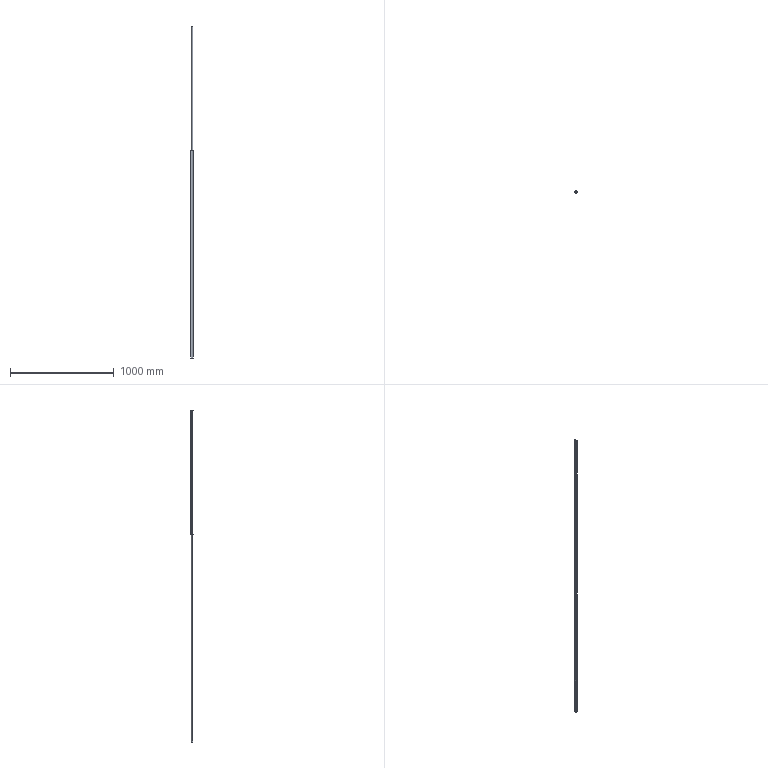Component | SolidWorks | 12ATransverseStraighteningPlatePart-2_12A10_Steel_Rib-1 | 4 solids | 16 faces | box 24 x 27 x 3200 mm | volume 723823 mm3 | cylinder 8 | plane 8 | commonest cylinder face diameters 12 x8
build123d program:
from build123d import *

# Parameters (mm, degrees)
SKETCH1_R             = 6
BOSS_EXTRUDE1_DEPTH   = 1200
BOSS_EXTRUDE1_2_DEPTH = 1200
SKETCH3_R             = 6
BOSS_EXTRUDE2_DEPTH   = 2000
SKETCH4_R             = 6
BOSS_EXTRUDE4_DEPTH   = 2000


with BuildPart() as part:
    # Sketch1 → Boss-Extrude1 (new body)
    with BuildSketch(Plane(origin=(0, 0, 0), x_dir=(1, 0, 0), z_dir=(0, 1, 0))):
        with Locations(Location((0, 0, 0), (0, 0, 270))):
            Circle(SKETCH1_R)
    extrude(amount=BOSS_EXTRUDE1_DEPTH)


with BuildPart() as body_2:
    # Sketch1 → Boss-Extrude1 2 (new body)
    with BuildSketch(Plane(origin=(0, 0, 0), x_dir=(1, 0, 0), z_dir=(0, 1, 0))):
        with Locations(Location((15, 0, 0), (0, 0, 270))):
            Circle(SKETCH1_R)
    extrude(amount=BOSS_EXTRUDE1_2_DEPTH)


with BuildPart() as body_3:
    # Sketch3 → Boss-Extrude2 (new body)
    with BuildSketch(Plane.XZ.offset(-1200)):
        with Locations(Location((7.5, -6, 0), (0, 0, 270))):
            Circle(SKETCH3_R)
    extrude(amount=-BOSS_EXTRUDE2_DEPTH)


with BuildPart() as body_4:
    # Sketch4 → Boss-Extrude4 (new body)
    with BuildSketch(Plane.XZ.offset(-1200)):
        with Locations(Location((7.5, 6, 0), (0, 0, 270))):
            Circle(SKETCH4_R)
    extrude(amount=-BOSS_EXTRUDE4_DEPTH)


solid = Compound([part.part, body_2.part, body_3.part, body_4.part])

# Placed as in the assembly
solid = solid.moved(Location((159.367, 112.46, 566), (-90, 90, 0)))
STEP:
#1=COLOUR_RGB('',0.7922,0.8196,0.9333);
#2=FILL_AREA_STYLE_COLOUR('',#1);
#3=FILL_AREA_STYLE('',(#2));
#4=SURFACE_STYLE_FILL_AREA(#3);
#5=SURFACE_SIDE_STYLE('',(#4));
#6=SURFACE_STYLE_USAGE(.BOTH.,#5);
#7=PRESENTATION_STYLE_ASSIGNMENT((#6));
#8=CARTESIAN_POINT('',(6.274,4.132,-103.701));
#9=VERTEX_POINT('',#8);
#10=CARTESIAN_POINT('',(6.747,4.132,-103.701));
#11=VERTEX_POINT('',#10);
#12=CARTESIAN_POINT('',(6.511,4.132,-103.701));
#13=DIRECTION('',(0.,0.,1.));
#14=DIRECTION('',(-1.,-0.,0.));
#15=AXIS2_PLACEMENT_3D('',#12,#13,#14);
#16=CIRCLE('',#15,0.2362);
#17=EDGE_CURVE('',#9,#11,#16,.T.);
#18=ORIENTED_EDGE('',*,*,#17,.T.);
#19=CARTESIAN_POINT('',(6.747,4.132,-24.961));
#20=VERTEX_POINT('',#19);
#21=CARTESIAN_POINT('',(6.747,4.132,-103.701));
#22=DIRECTION('',(0.,0.,1.));
#23=VECTOR('',#22,39.37);
#24=LINE('',#21,#23);
#25=EDGE_CURVE('',#11,#20,#24,.T.);
#26=ORIENTED_EDGE('',*,*,#25,.T.);
#27=CARTESIAN_POINT('',(6.274,4.132,-24.961));
#28=VERTEX_POINT('',#27);
#29=CARTESIAN_POINT('',(6.511,4.132,-24.961));
#30=DIRECTION('',(0.,0.,1.));
#31=DIRECTION('',(-1.,-0.,0.));
#32=AXIS2_PLACEMENT_3D('',#29,#30,#31);
#33=CIRCLE('',#32,0.2362);
#34=EDGE_CURVE('',#28,#20,#33,.T.);
#35=ORIENTED_EDGE('',*,*,#34,.F.);
#36=CARTESIAN_POINT('',(6.274,4.132,-103.701));
#37=DIRECTION('',(0.,0.,1.));
#38=VECTOR('',#37,39.37);
#39=LINE('',#36,#38);
#40=EDGE_CURVE('',#9,#28,#39,.T.);
#41=ORIENTED_EDGE('',*,*,#40,.F.);
#42=EDGE_LOOP('',(#18,#26,#35,#41));
#43=FACE_OUTER_BOUND('',#42,.T.);
#44=CARTESIAN_POINT('',(6.511,4.132,-103.701));
#45=DIRECTION('',(0.,0.,1.));
#46=DIRECTION('',(-1.,-0.,0.));
#47=AXIS2_PLACEMENT_3D('',#44,#45,#46);
#48=CYLINDRICAL_SURFACE('',#47,0.2362);
#49=ADVANCED_FACE('',(#43),#48,.T.);
#50=ORIENTED_EDGE('',*,*,#25,.F.);
#51=CARTESIAN_POINT('',(6.511,4.132,-103.701));
#52=DIRECTION('',(0.,0.,1.));
#53=DIRECTION('',(-1.,-0.,0.));
#54=AXIS2_PLACEMENT_3D('',#51,#52,#53);
#55=CIRCLE('',#54,0.2362);
#56=EDGE_CURVE('',#11,#9,#55,.T.);
#57=ORIENTED_EDGE('',*,*,#56,.T.);
#58=ORIENTED_EDGE('',*,*,#40,.T.);
#59=CARTESIAN_POINT('',(6.511,4.132,-24.961));
#60=DIRECTION('',(0.,0.,1.));
#61=DIRECTION('',(-1.,-0.,0.));
#62=AXIS2_PLACEMENT_3D('',#59,#60,#61);
#63=CIRCLE('',#62,0.2362);
#64=EDGE_CURVE('',#20,#28,#63,.T.);
#65=ORIENTED_EDGE('',*,*,#64,.F.);
#66=EDGE_LOOP('',(#50,#57,#58,#65));
#67=FACE_OUTER_BOUND('',#66,.T.);
#68=CARTESIAN_POINT('',(6.511,4.132,-103.701));
#69=DIRECTION('',(0.,0.,1.));
#70=DIRECTION('',(-1.,-0.,0.));
#71=AXIS2_PLACEMENT_3D('',#68,#69,#70);
#72=CYLINDRICAL_SURFACE('',#71,0.2362);
#73=ADVANCED_FACE('',(#67),#72,.T.);
#74=ORIENTED_EDGE('',*,*,#17,.F.);
#75=ORIENTED_EDGE('',*,*,#56,.F.);
#76=EDGE_LOOP('',(#74,#75));
#77=FACE_OUTER_BOUND('',#76,.T.);
#78=CARTESIAN_POINT('',(6.511,4.132,-103.701));
#79=DIRECTION('',(0.,0.,1.));
#80=DIRECTION('',(-1.,-0.,0.));
#81=AXIS2_PLACEMENT_3D('',#78,#79,#80);
#82=PLANE('',#81);
#83=ADVANCED_FACE('',(#77),#82,.F.);
#84=ORIENTED_EDGE('',*,*,#34,.T.);
#85=ORIENTED_EDGE('',*,*,#64,.T.);
#86=EDGE_LOOP('',(#84,#85));
#87=FACE_OUTER_BOUND('',#86,.T.);
#88=CARTESIAN_POINT('',(6.511,4.132,-24.961));
#89=DIRECTION('',(0.,0.,1.));
#90=DIRECTION('',(-1.,-0.,0.));
#91=AXIS2_PLACEMENT_3D('',#88,#89,#90);
#92=PLANE('',#91);
#93=ADVANCED_FACE('',(#87),#92,.T.);
#94=CLOSED_SHELL('',(#49,#73,#83,#93));
#95=MANIFOLD_SOLID_BREP('',#94);
#96=STYLED_ITEM('',(#7),#95);
#97=(LENGTH_UNIT()NAMED_UNIT(*)SI_UNIT($,.METRE.));
#98=LENGTH_MEASURE_WITH_UNIT(LENGTH_MEASURE(0.0254),#97);
#99=DIMENSIONAL_EXPONENTS(1.,0.,0.,0.,0.,0.,0.);
#100=(CONVERSION_BASED_UNIT('',#98)LENGTH_UNIT()NAMED_UNIT(#99));
#101=UNCERTAINTY_MEASURE_WITH_UNIT(LENGTH_MEASURE(0.00001),#100,'','');
#102=(NAMED_UNIT(*)PLANE_ANGLE_UNIT()SI_UNIT($,.RADIAN.));
#103=(NAMED_UNIT(*)SI_UNIT($,.STERADIAN.)SOLID_ANGLE_UNIT());
#104=(GEOMETRIC_REPRESENTATION_CONTEXT(3)GLOBAL_UNCERTAINTY_ASSIGNED_CONTEXT((#101))GLOBAL_UNIT_ASSIGNED_CONTEXT((#100,#102,#103))REPRESENTATION_CONTEXT('',''));
#105=MECHANICAL_DESIGN_GEOMETRIC_PRESENTATION_REPRESENTATION('',(#96),#104);
#106=COLOUR_RGB('',0.7922,0.8196,0.9333);
#107=FILL_AREA_STYLE_COLOUR('',#106);
#108=FILL_AREA_STYLE('',(#107));
#109=SURFACE_STYLE_FILL_AREA(#108);
#110=SURFACE_SIDE_STYLE('',(#109));
#111=SURFACE_STYLE_USAGE(.BOTH.,#110);
#112=PRESENTATION_STYLE_ASSIGNMENT((#111));
#113=CARTESIAN_POINT('',(5.802,4.132,-103.701));
#114=VERTEX_POINT('',#113);
#115=CARTESIAN_POINT('',(6.274,4.132,-103.701));
#116=VERTEX_POINT('',#115);
#117=CARTESIAN_POINT('',(6.038,4.132,-103.701));
#118=DIRECTION('',(0.,0.,1.));
#119=DIRECTION('',(-1.,-0.,0.));
#120=AXIS2_PLACEMENT_3D('',#117,#118,#119);
#121=CIRCLE('',#120,0.2362);
#122=EDGE_CURVE('',#114,#116,#121,.T.);
#123=ORIENTED_EDGE('',*,*,#122,.T.);
#124=CARTESIAN_POINT('',(6.274,4.132,-24.961));
#125=VERTEX_POINT('',#124);
#126=CARTESIAN_POINT('',(6.274,4.132,-103.701));
#127=DIRECTION('',(0.,0.,1.));
#128=VECTOR('',#127,39.37);
#129=LINE('',#126,#128);
#130=EDGE_CURVE('',#116,#125,#129,.T.);
#131=ORIENTED_EDGE('',*,*,#130,.T.);
#132=CARTESIAN_POINT('',(5.802,4.132,-24.961));
#133=VERTEX_POINT('',#132);
#134=CARTESIAN_POINT('',(6.038,4.132,-24.961));
#135=DIRECTION('',(0.,0.,1.));
#136=DIRECTION('',(-1.,-0.,0.));
#137=AXIS2_PLACEMENT_3D('',#134,#135,#136);
#138=CIRCLE('',#137,0.2362);
#139=EDGE_CURVE('',#133,#125,#138,.T.);
#140=ORIENTED_EDGE('',*,*,#139,.F.);
#141=CARTESIAN_POINT('',(5.802,4.132,-103.701));
#142=DIRECTION('',(0.,0.,1.));
#143=VECTOR('',#142,39.37);
#144=LINE('',#141,#143);
#145=EDGE_CURVE('',#114,#133,#144,.T.);
#146=ORIENTED_EDGE('',*,*,#145,.F.);
#147=EDGE_LOOP('',(#123,#131,#140,#146));
#148=FACE_OUTER_BOUND('',#147,.T.);
#149=CARTESIAN_POINT('',(6.038,4.132,-103.701));
#150=DIRECTION('',(0.,0.,1.));
#151=DIRECTION('',(-1.,-0.,0.));
#152=AXIS2_PLACEMENT_3D('',#149,#150,#151);
#153=CYLINDRICAL_SURFACE('',#152,0.2362);
#154=ADVANCED_FACE('',(#148),#153,.T.);
#155=ORIENTED_EDGE('',*,*,#130,.F.);
#156=CARTESIAN_POINT('',(6.038,4.132,-103.701));
#157=DIRECTION('',(0.,0.,1.));
#158=DIRECTION('',(-1.,-0.,0.));
#159=AXIS2_PLACEMENT_3D('',#156,#157,#158);
#160=CIRCLE('',#159,0.2362);
#161=EDGE_CURVE('',#116,#114,#160,.T.);
#162=ORIENTED_EDGE('',*,*,#161,.T.);
#163=ORIENTED_EDGE('',*,*,#145,.T.);
#164=CARTESIAN_POINT('',(6.038,4.132,-24.961));
#165=DIRECTION('',(0.,0.,1.));
#166=DIRECTION('',(-1.,-0.,0.));
#167=AXIS2_PLACEMENT_3D('',#164,#165,#166);
#168=CIRCLE('',#167,0.2362);
#169=EDGE_CURVE('',#125,#133,#168,.T.);
#170=ORIENTED_EDGE('',*,*,#169,.F.);
#171=EDGE_LOOP('',(#155,#162,#163,#170));
#172=FACE_OUTER_BOUND('',#171,.T.);
#173=CARTESIAN_POINT('',(6.038,4.132,-103.701));
#174=DIRECTION('',(0.,0.,1.));
#175=DIRECTION('',(-1.,-0.,0.));
#176=AXIS2_PLACEMENT_3D('',#173,#174,#175);
#177=CYLINDRICAL_SURFACE('',#176,0.2362);
#178=ADVANCED_FACE('',(#172),#177,.T.);
#179=ORIENTED_EDGE('',*,*,#122,.F.);
#180=ORIENTED_EDGE('',*,*,#161,.F.);
#181=EDGE_LOOP('',(#179,#180));
#182=FACE_OUTER_BOUND('',#181,.T.);
#183=CARTESIAN_POINT('',(6.038,4.132,-103.701));
#184=DIRECTION('',(0.,0.,1.));
#185=DIRECTION('',(-1.,-0.,0.));
#186=AXIS2_PLACEMENT_3D('',#183,#184,#185);
#187=PLANE('',#186);
#188=ADVANCED_FACE('',(#182),#187,.F.);
#189=ORIENTED_EDGE('',*,*,#139,.T.);
#190=ORIENTED_EDGE('',*,*,#169,.T.);
#191=EDGE_LOOP('',(#189,#190));
#192=FACE_OUTER_BOUND('',#191,.T.);
#193=CARTESIAN_POINT('',(6.038,4.132,-24.961));
#194=DIRECTION('',(0.,0.,1.));
#195=DIRECTION('',(-1.,-0.,0.));
#196=AXIS2_PLACEMENT_3D('',#193,#194,#195);
#197=PLANE('',#196);
#198=ADVANCED_FACE('',(#192),#197,.T.);
#199=CLOSED_SHELL('',(#154,#178,#188,#198));
#200=MANIFOLD_SOLID_BREP('',#199);
#201=STYLED_ITEM('',(#112),#200);
#202=PRESENTATION_LAYER_ASSIGNMENT('','',(#201));
#203=(LENGTH_UNIT()NAMED_UNIT(*)SI_UNIT($,.METRE.));
#204=LENGTH_MEASURE_WITH_UNIT(LENGTH_MEASURE(0.0254),#203);
#205=DIMENSIONAL_EXPONENTS(1.,0.,0.,0.,0.,0.,0.);
#206=(CONVERSION_BASED_UNIT('',#204)LENGTH_UNIT()NAMED_UNIT(#205));
#207=UNCERTAINTY_MEASURE_WITH_UNIT(LENGTH_MEASURE(0.00001),#206,'','');
#208=(NAMED_UNIT(*)PLANE_ANGLE_UNIT()SI_UNIT($,.RADIAN.));
#209=(NAMED_UNIT(*)SI_UNIT($,.STERADIAN.)SOLID_ANGLE_UNIT());
#210=(GEOMETRIC_REPRESENTATION_CONTEXT(3)GLOBAL_UNCERTAINTY_ASSIGNED_CONTEXT((#207))GLOBAL_UNIT_ASSIGNED_CONTEXT((#206,#208,#209))REPRESENTATION_CONTEXT('',''));
#211=MECHANICAL_DESIGN_GEOMETRIC_PRESENTATION_REPRESENTATION('',(#201),#210);
#212=COLOUR_RGB('',0.7922,0.8196,0.9333);
#213=FILL_AREA_STYLE_COLOUR('',#212);
#214=FILL_AREA_STYLE('',(#213));
#215=SURFACE_STYLE_FILL_AREA(#214);
#216=SURFACE_SIDE_STYLE('',(#215));
#217=SURFACE_STYLE_USAGE(.BOTH.,#216);
#218=PRESENTATION_STYLE_ASSIGNMENT((#217));
#219=CARTESIAN_POINT('',(6.511,4.428,-24.961));
#220=VERTEX_POINT('',#219);
#221=CARTESIAN_POINT('',(6.038,4.428,-24.961));
#222=VERTEX_POINT('',#221);
#223=CARTESIAN_POINT('',(6.274,4.428,-24.961));
#224=DIRECTION('',(-0.,-0.,-1.));
#225=DIRECTION('',(1.,0.,0.));
#226=AXIS2_PLACEMENT_3D('',#223,#224,#225);
#227=CIRCLE('',#226,0.2362);
#228=EDGE_CURVE('',#220,#222,#227,.T.);
#229=ORIENTED_EDGE('',*,*,#228,.F.);
#230=CARTESIAN_POINT('',(6.511,4.428,22.283));
#231=VERTEX_POINT('',#230);
#232=CARTESIAN_POINT('',(6.511,4.428,-24.961));
#233=DIRECTION('',(0.,0.,1.));
#234=VECTOR('',#233,39.37);
#235=LINE('',#232,#234);
#236=EDGE_CURVE('',#220,#231,#235,.T.);
#237=ORIENTED_EDGE('',*,*,#236,.T.);
#238=CARTESIAN_POINT('',(6.038,4.428,22.283));
#239=VERTEX_POINT('',#238);
#240=CARTESIAN_POINT('',(6.274,4.428,22.283));
#241=DIRECTION('',(-0.,-0.,-1.));
#242=DIRECTION('',(1.,0.,0.));
#243=AXIS2_PLACEMENT_3D('',#240,#241,#242);
#244=CIRCLE('',#243,0.2362);
#245=EDGE_CURVE('',#231,#239,#244,.T.);
#246=ORIENTED_EDGE('',*,*,#245,.T.);
#247=CARTESIAN_POINT('',(6.038,4.428,-24.961));
#248=DIRECTION('',(0.,0.,1.));
#249=VECTOR('',#248,39.37);
#250=LINE('',#247,#249);
#251=EDGE_CURVE('',#222,#239,#250,.T.);
#252=ORIENTED_EDGE('',*,*,#251,.F.);
#253=EDGE_LOOP('',(#229,#237,#246,#252));
#254=FACE_OUTER_BOUND('',#253,.T.);
#255=CARTESIAN_POINT('',(6.274,4.428,-24.961));
#256=DIRECTION('',(0.,0.,1.));
#257=DIRECTION('',(-1.,-0.,0.));
#258=AXIS2_PLACEMENT_3D('',#255,#256,#257);
#259=CYLINDRICAL_SURFACE('',#258,0.2362);
#260=ADVANCED_FACE('',(#254),#259,.T.);
#261=ORIENTED_EDGE('',*,*,#236,.F.);
#262=CARTESIAN_POINT('',(6.274,4.428,-24.961));
#263=DIRECTION('',(-0.,-0.,-1.));
#264=DIRECTION('',(1.,0.,0.));
#265=AXIS2_PLACEMENT_3D('',#262,#263,#264);
#266=CIRCLE('',#265,0.2362);
#267=EDGE_CURVE('',#222,#220,#266,.T.);
#268=ORIENTED_EDGE('',*,*,#267,.F.);
#269=ORIENTED_EDGE('',*,*,#251,.T.);
#270=CARTESIAN_POINT('',(6.274,4.428,22.283));
#271=DIRECTION('',(-0.,-0.,-1.));
#272=DIRECTION('',(1.,0.,0.));
#273=AXIS2_PLACEMENT_3D('',#270,#271,#272);
#274=CIRCLE('',#273,0.2362);
#275=EDGE_CURVE('',#239,#231,#274,.T.);
#276=ORIENTED_EDGE('',*,*,#275,.T.);
#277=EDGE_LOOP('',(#261,#268,#269,#276));
#278=FACE_OUTER_BOUND('',#277,.T.);
#279=CARTESIAN_POINT('',(6.274,4.428,-24.961));
#280=DIRECTION('',(0.,0.,1.));
#281=DIRECTION('',(-1.,-0.,0.));
#282=AXIS2_PLACEMENT_3D('',#279,#280,#281);
#283=CYLINDRICAL_SURFACE('',#282,0.2362);
#284=ADVANCED_FACE('',(#278),#283,.T.);
#285=ORIENTED_EDGE('',*,*,#267,.T.);
#286=ORIENTED_EDGE('',*,*,#228,.T.);
#287=EDGE_LOOP('',(#285,#286));
#288=FACE_OUTER_BOUND('',#287,.T.);
#289=CARTESIAN_POINT('',(6.274,4.428,-24.961));
#290=DIRECTION('',(-0.,-0.,-1.));
#291=DIRECTION('',(1.,0.,-0.));
#292=AXIS2_PLACEMENT_3D('',#289,#290,#291);
#293=PLANE('',#292);
#294=ADVANCED_FACE('',(#288),#293,.T.);
#295=ORIENTED_EDGE('',*,*,#275,.F.);
#296=ORIENTED_EDGE('',*,*,#245,.F.);
#297=EDGE_LOOP('',(#295,#296));
#298=FACE_OUTER_BOUND('',#297,.T.);
#299=CARTESIAN_POINT('',(6.274,4.428,22.283));
#300=DIRECTION('',(-0.,-0.,-1.));
#301=DIRECTION('',(1.,0.,-0.));
#302=AXIS2_PLACEMENT_3D('',#299,#300,#301);
#303=PLANE('',#302);
#304=ADVANCED_FACE('',(#298),#303,.F.);
#305=CLOSED_SHELL('',(#260,#284,#294,#304));
#306=MANIFOLD_SOLID_BREP('',#305);
#307=STYLED_ITEM('',(#218),#306);
#308=(LENGTH_UNIT()NAMED_UNIT(*)SI_UNIT($,.METRE.));
#309=LENGTH_MEASURE_WITH_UNIT(LENGTH_MEASURE(0.0254),#308);
#310=DIMENSIONAL_EXPONENTS(1.,0.,0.,0.,0.,0.,0.);
#311=(CONVERSION_BASED_UNIT('',#309)LENGTH_UNIT()NAMED_UNIT(#310));
#312=UNCERTAINTY_MEASURE_WITH_UNIT(LENGTH_MEASURE(0.00001),#311,'','');
#313=(NAMED_UNIT(*)PLANE_ANGLE_UNIT()SI_UNIT($,.RADIAN.));
#314=(NAMED_UNIT(*)SI_UNIT($,.STERADIAN.)SOLID_ANGLE_UNIT());
#315=(GEOMETRIC_REPRESENTATION_CONTEXT(3)GLOBAL_UNCERTAINTY_ASSIGNED_CONTEXT((#312))GLOBAL_UNIT_ASSIGNED_CONTEXT((#311,#313,#314))REPRESENTATION_CONTEXT('',''));
#316=MECHANICAL_DESIGN_GEOMETRIC_PRESENTATION_REPRESENTATION('',(#307),#315);
#317=PRESENTATION_LAYER_ASSIGNMENT('','',(#96));
#318=COLOUR_RGB('',0.7922,0.8196,0.9333);
#319=FILL_AREA_STYLE_COLOUR('',#318);
#320=FILL_AREA_STYLE('',(#319));
#321=SURFACE_STYLE_FILL_AREA(#320);
#322=SURFACE_SIDE_STYLE('',(#321));
#323=SURFACE_STYLE_USAGE(.BOTH.,#322);
#324=PRESENTATION_STYLE_ASSIGNMENT((#323));
#325=CARTESIAN_POINT('',(6.511,3.837,-24.961));
#326=VERTEX_POINT('',#325);
#327=CARTESIAN_POINT('',(6.038,3.837,-24.961));
#328=VERTEX_POINT('',#327);
#329=CARTESIAN_POINT('',(6.274,3.837,-24.961));
#330=DIRECTION('',(-0.,-0.,-1.));
#331=DIRECTION('',(1.,0.,0.));
#332=AXIS2_PLACEMENT_3D('',#329,#330,#331);
#333=CIRCLE('',#332,0.2362);
#334=EDGE_CURVE('',#326,#328,#333,.T.);
#335=ORIENTED_EDGE('',*,*,#334,.F.);
#336=CARTESIAN_POINT('',(6.511,3.837,22.283));
#337=VERTEX_POINT('',#336);
#338=CARTESIAN_POINT('',(6.511,3.837,-24.961));
#339=DIRECTION('',(0.,0.,1.));
#340=VECTOR('',#339,39.37);
#341=LINE('',#338,#340);
#342=EDGE_CURVE('',#326,#337,#341,.T.);
#343=ORIENTED_EDGE('',*,*,#342,.T.);
#344=CARTESIAN_POINT('',(6.038,3.837,22.283));
#345=VERTEX_POINT('',#344);
#346=CARTESIAN_POINT('',(6.274,3.837,22.283));
#347=DIRECTION('',(-0.,-0.,-1.));
#348=DIRECTION('',(1.,0.,0.));
#349=AXIS2_PLACEMENT_3D('',#346,#347,#348);
#350=CIRCLE('',#349,0.2362);
#351=EDGE_CURVE('',#337,#345,#350,.T.);
#352=ORIENTED_EDGE('',*,*,#351,.T.);
#353=CARTESIAN_POINT('',(6.038,3.837,-24.961));
#354=DIRECTION('',(0.,0.,1.));
#355=VECTOR('',#354,39.37);
#356=LINE('',#353,#355);
#357=EDGE_CURVE('',#328,#345,#356,.T.);
#358=ORIENTED_EDGE('',*,*,#357,.F.);
#359=EDGE_LOOP('',(#335,#343,#352,#358));
#360=FACE_OUTER_BOUND('',#359,.T.);
#361=CARTESIAN_POINT('',(6.274,3.837,-24.961));
#362=DIRECTION('',(0.,0.,1.));
#363=DIRECTION('',(-1.,-0.,0.));
#364=AXIS2_PLACEMENT_3D('',#361,#362,#363);
#365=CYLINDRICAL_SURFACE('',#364,0.2362);
#366=ADVANCED_FACE('',(#360),#365,.T.);
#367=ORIENTED_EDGE('',*,*,#342,.F.);
#368=CARTESIAN_POINT('',(6.274,3.837,-24.961));
#369=DIRECTION('',(-0.,-0.,-1.));
#370=DIRECTION('',(1.,0.,0.));
#371=AXIS2_PLACEMENT_3D('',#368,#369,#370);
#372=CIRCLE('',#371,0.2362);
#373=EDGE_CURVE('',#328,#326,#372,.T.);
#374=ORIENTED_EDGE('',*,*,#373,.F.);
#375=ORIENTED_EDGE('',*,*,#357,.T.);
#376=CARTESIAN_POINT('',(6.274,3.837,22.283));
#377=DIRECTION('',(-0.,-0.,-1.));
#378=DIRECTION('',(1.,0.,0.));
#379=AXIS2_PLACEMENT_3D('',#376,#377,#378);
#380=CIRCLE('',#379,0.2362);
#381=EDGE_CURVE('',#345,#337,#380,.T.);
#382=ORIENTED_EDGE('',*,*,#381,.T.);
#383=EDGE_LOOP('',(#367,#374,#375,#382));
#384=FACE_OUTER_BOUND('',#383,.T.);
#385=CARTESIAN_POINT('',(6.274,3.837,-24.961));
#386=DIRECTION('',(0.,0.,1.));
#387=DIRECTION('',(-1.,-0.,0.));
#388=AXIS2_PLACEMENT_3D('',#385,#386,#387);
#389=CYLINDRICAL_SURFACE('',#388,0.2362);
#390=ADVANCED_FACE('',(#384),#389,.T.);
#391=ORIENTED_EDGE('',*,*,#373,.T.);
#392=ORIENTED_EDGE('',*,*,#334,.T.);
#393=EDGE_LOOP('',(#391,#392));
#394=FACE_OUTER_BOUND('',#393,.T.);
#395=CARTESIAN_POINT('',(6.274,3.837,-24.961));
#396=DIRECTION('',(-0.,-0.,-1.));
#397=DIRECTION('',(1.,0.,-0.));
#398=AXIS2_PLACEMENT_3D('',#395,#396,#397);
#399=PLANE('',#398);
#400=ADVANCED_FACE('',(#394),#399,.T.);
#401=ORIENTED_EDGE('',*,*,#381,.F.);
#402=ORIENTED_EDGE('',*,*,#351,.F.);
#403=EDGE_LOOP('',(#401,#402));
#404=FACE_OUTER_BOUND('',#403,.T.);
#405=CARTESIAN_POINT('',(6.274,3.837,22.283));
#406=DIRECTION('',(-0.,-0.,-1.));
#407=DIRECTION('',(1.,0.,-0.));
#408=AXIS2_PLACEMENT_3D('',#405,#406,#407);
#409=PLANE('',#408);
#410=ADVANCED_FACE('',(#404),#409,.F.);
#411=CLOSED_SHELL('',(#366,#390,#400,#410));
#412=MANIFOLD_SOLID_BREP('',#411);
#413=STYLED_ITEM('',(#324),#412);
#414=PRESENTATION_LAYER_ASSIGNMENT('','',(#413));
#415=(LENGTH_UNIT()NAMED_UNIT(*)SI_UNIT($,.METRE.));
#416=LENGTH_MEASURE_WITH_UNIT(LENGTH_MEASURE(0.0254),#415);
#417=DIMENSIONAL_EXPONENTS(1.,0.,0.,0.,0.,0.,0.);
#418=(CONVERSION_BASED_UNIT('',#416)LENGTH_UNIT()NAMED_UNIT(#417));
#419=UNCERTAINTY_MEASURE_WITH_UNIT(LENGTH_MEASURE(0.00001),#418,'','');
#420=(NAMED_UNIT(*)PLANE_ANGLE_UNIT()SI_UNIT($,.RADIAN.));
#421=(NAMED_UNIT(*)SI_UNIT($,.STERADIAN.)SOLID_ANGLE_UNIT());
#422=(GEOMETRIC_REPRESENTATION_CONTEXT(3)GLOBAL_UNCERTAINTY_ASSIGNED_CONTEXT((#419))GLOBAL_UNIT_ASSIGNED_CONTEXT((#418,#420,#421))REPRESENTATION_CONTEXT('',''));
#423=MECHANICAL_DESIGN_GEOMETRIC_PRESENTATION_REPRESENTATION('',(#413),#422);
#424=CARTESIAN_POINT('',(0.,0.,0.));
#425=DIRECTION('',(0.,0.,1.));
#426=DIRECTION('',(1.,0.,0.));
#427=AXIS2_PLACEMENT_3D('',#424,#425,#426);
#428=(LENGTH_UNIT()NAMED_UNIT(*)SI_UNIT($,.METRE.));
#429=LENGTH_MEASURE_WITH_UNIT(LENGTH_MEASURE(0.0254),#428);
#430=DIMENSIONAL_EXPONENTS(1.,0.,0.,0.,0.,0.,0.);
#431=(CONVERSION_BASED_UNIT('',#429)LENGTH_UNIT()NAMED_UNIT(#430));
#432=UNCERTAINTY_MEASURE_WITH_UNIT(LENGTH_MEASURE(0.00001),#431,'','');
#433=(NAMED_UNIT(*)PLANE_ANGLE_UNIT()SI_UNIT($,.RADIAN.));
#434=(NAMED_UNIT(*)SI_UNIT($,.STERADIAN.)SOLID_ANGLE_UNIT());
#435=(GEOMETRIC_REPRESENTATION_CONTEXT(3)GLOBAL_UNCERTAINTY_ASSIGNED_CONTEXT((#432))GLOBAL_UNIT_ASSIGNED_CONTEXT((#431,#433,#434))REPRESENTATION_CONTEXT('',''));
#436=ADVANCED_BREP_SHAPE_REPRESENTATION('',(#412,#306,#95,#200,#427),#435);
#437=PRESENTATION_LAYER_ASSIGNMENT('','',(#307));